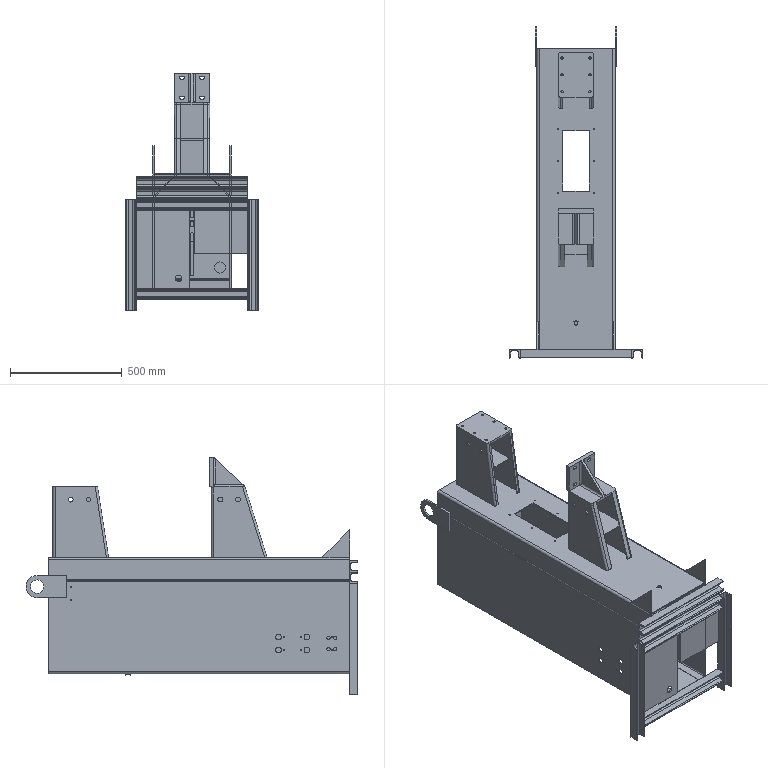Assembly | SolidWorks | mm | 24 component files | 27 solids | 480 faces | box 600 x 1487 x 1065 mm | volume 20129983 mm3 | plane 256 | cylinder 218 | cone 4 | torus 2 | commonest cylinder face diameters 5 x30 10 x27 14 x26 20 x17 7 x14 60 x12 50 x12 10.2 x12
Bill of materials:
001LowerConnectingPlate | 1 | Plain Carbon Steel | Flat rectangular plate, roughly 2:1 aspect ratio, with one large round through-hole and one small round through-hole offset toward one side.
001ReinforcingRib | 2 | Plain Carbon Steel | Thin flat plate with a right-triangle outline (two equal legs at 90 degrees), no visible holes.
001UpperConnectingPlate | 1 | Plain Carbon Steel | Plain flat rectangular plate, roughly 2:1 aspect ratio, with no holes or cutouts.
002FrameBasePanel | 1 | Plain Carbon Steel | Thin flat rectangular plate (portrait proportion) with a single round through-hole near one corner.
002FrameBasePanel2 | 1 | Plain Carbon Steel | Thin flat rectangular plate, slightly wider than tall, with no visible holes or cutouts.
hot-rolled steel channel gb | 6 |  | Straight prismatic channel (C-shaped) profile: a flat web with two flanges whose inner faces taper toward the tips, with filleted inner corners and rounded flange tips.
003FrameFrontWeldingPlate | 1 | Plain Carbon Steel | Bent sheet-metal U-shaped cover/channel: flat top web with two downturned side flanges, a central rectangular cutout, two round holes on either side of it, one small hole near one end, and several tiny point features around the cutout.
004FrameSheet-MetalA | 1 | Plain Carbon Steel | Long bent sheet-metal panel: tall flat web with an inclined top flange and a short bottom return flange, with a small rolled or hooked feature at the bottom bend; a cluster of round holes near one end and two tiny holes near the other end.
005FrameSheet-MetalB | 1 | Plain Carbon Steel | Long bent sheet-metal panel with a tall flat web, an inclined top flange, and a short bottom return flange; one round through-hole and two tiny holes/marks in the web.
006TransformerBasePlate | 1 | Plain Carbon Steel | Sheet-metal bracket plate with chamfered upper corners (pentagon-like outline) and a short bent flange along the bottom edge; four round holes near the corners and two collinear slots along the vertical centerline.
007PartitionPlate | 1 | Plain Carbon Steel | Flat thin plate with chamfered upper corners (pentagon-like outline) and four round through-holes: two near the top and two near the bottom corners.
008FrameTopCoverPlate | 1 | Plain Carbon Steel | Very thin flat rectangular plate (portrait proportion) with slightly rounded corners and two small round holes near the top corners.
009LiftingLug | 2 | Plain Carbon Steel | Flat plate tab of constant thickness. One end is square and the other end is a full semicircle. A single through-hole sits concentric with the rounded end.
010MachineHeadWeldedPart | 1 | Plain Carbon Steel | Formed hollow sheet-metal housing or stand shape. It has a flat top panel with six small holes and side walls that taper and flare outward toward the bottom. Two opposite sides are open below a cross panel, which leaves leg-like wall sections. Each side wall has one larger round hole near the top.
011FrameLowerElectrodeWeldedPart | 1 | Plain Carbon Steel | Bracket with a vertical rectangular mounting flange on top. The flange carries four slotted holes split by a central vertical rib or gusset. The rib slopes down to a tapered, formed channel body with two legs, an internal cross panel, and round holes in the side walls.
hot-rolled equal angle gb | 2 |  | Straight, constant-section angle profile (L-section) with two legs of roughly equal length. It has a root fillet at the inside corner and small rounded tips on the legs. Both ends are cut square.
Mates:
1. distance | 010MachineHeadWeldedPart-1 face at (210, 1367, 320) dir (0, 1, 0) | 011FrameLowerElectrodeWeldedPart-1 face at (210, 657, 320) dir (0, 1, 0)
2. distance | 007PartitionPlate-2 face at (299, 1207, -306) dir (0, 1, 0) | 006TransformerBasePlate-1 face at (-39, 647, -481) dir (0, 1, 0)
3. distance | hot-rolled equal angle gb-1 face at (160, 187, -195) dir (0, -1, 0) | hot-rolled equal angle gb-6 face at (160, 537, -195) dir (0, -1, 0)
4. coincident | 011FrameLowerElectrodeWeldedPart-1 face at (210, 407, 0) dir (0, 0, -1) | 010MachineHeadWeldedPart-1 face at (210, 1117, 0) dir (0, 0, -1)
5. coincident | 011FrameLowerElectrodeWeldedPart-1 face at (50, 667, 320) dir (-1, 0, 0) | 010MachineHeadWeldedPart-1 face at (50, 1367, 0) dir (-1, 0, 0)
6. coincident | 006TransformerBasePlate-1 face at (197.5, 647, -6) dir (0, 0, 1) | 007PartitionPlate-2 face at (62.5, 1202, -6) dir (0, 0, 1)
7. distance | hot-rolled equal angle gb-1 face at (160, 187, -195) dir (0, -1, 0) | 002FrameBaseAssembly-1/002FrameBasePanel-1 face at (-120, 37, -515) dir (0, 1, 0)
8. coincident | hot-rolled equal angle gb-1 face at (-40, 189, -196) dir (-1, 0, 0) | hot-rolled equal angle gb-6 face at (-40, 539, -196) dir (-1, 0, 0)
9. coincident | hot-rolled equal angle gb-1 face at (160, 187, -215) dir (0, 0, -1) | hot-rolled equal angle gb-6 face at (160, 537, -215) dir (0, 0, -1)
10. distance | 006TransformerBasePlate-1 face at (-39, 647, -481) dir (0, 1, 0) | 002FrameBaseAssembly-1/002FrameBasePanel-1 face at (-120, 37, -515) dir (0, 1, 0)
11. coincident | 002FrameBaseAssembly-1/002FrameBasePanel-1 face at (-120, 37, -515) dir (0, 1, 0) | 001LowerConnectingPlate-1 face at (260, 37, -520) dir (0, -1, 0)
12. coincident | 003FrameFrontWeldingPlate-1 face at (-45, 1387, 0) dir (-1, 0, 0) | 001ReinforcingRib-1 face at (-45, 162, 0) dir (-1, 0, 0)
13. coincident | 002FrameBaseAssembly-1/002FrameBasePanel-1 face at (-120, 37, -515) dir (0, 1, 0) | 001ReinforcingRib-1 face at (-45, 37, 0) dir (0, -1, 0)
14. coincident | 003FrameFrontWeldingPlate-1 face at (-45, 1387, 0) dir (0, 0, 1) | 001ReinforcingRib-1 face at (-45, 162, 0) dir (0, 0, -1)
15. distance | 002FrameBaseAssembly-1/hot-rolled steel channel gb-5 face at (420.925, 37, -615) dir (0, 0, -1) | 005FrameSheet-MetalB-1 face at (-105, 1387, -520) dir (0, 0, -1)
16. coincident | 001UpperConnectingPlate-1 face at (260, 1387, -520) dir (0, 0, -1) | 001LowerConnectingPlate-1 face at (0, 162, -520) dir (0, 0, -1)
17. coincident | 004FrameSheet-MetalA-1 face at (0, 1526.253, -4.999) dir (1, 0, 0) | 001LowerConnectingPlate-1 face at (0, 37, -520) dir (-1, 0, 0)
18. coincident | 004FrameSheet-MetalA-1 face at (-40, 1387, -5) dir (1, 0, 0) | hot-rolled equal angle gb-1 face at (-40, 189, -196) dir (-1, 0, 0)
19. distance | 003FrameFrontWeldingPlate-1 face at (-45, 1387, -5) dir (0, 0, -1) | 006TransformerBasePlate-1 face at (197.5, 647, -6) dir (0, 0, 1)
20. distance | hot-rolled equal angle gb-6 edge at (160, 537, -215) dir (-1, 0, 0) | 004FrameSheet-MetalA-1 face at (-45, 1387, -515) dir (0, 0, 1)
21. coincident | 005FrameSheet-MetalB-1 face at (-105, 1387, -520) dir (0, 0, -1) | 001UpperConnectingPlate-1 face at (260, 1387, -520) dir (0, 0, -1)
22. coincident | 005FrameSheet-MetalB-1 face at (305, 1387, -520) dir (0, 1, 0) | 001UpperConnectingPlate-1 face at (0, 1387, -515) dir (0, 1, 0)
23. coincident | 004FrameSheet-MetalA-1 face at (0, 1526.253, -4.999) dir (1, 0, 0) | 001UpperConnectingPlate-1 face at (0, 1247, -515) dir (-1, 0, 0)
24. distance | 008FrameTopCoverPlate-1 face at (299, 1377, -515) dir (0, 1, 0) | 003FrameFrontWeldingPlate-1 face at (305, 1387, -100) dir (0, 1, 0)
25. coincident | 011FrameLowerElectrodeWeldedPart-1 face at (210, 407, 0) dir (0, 0, -1) | 003FrameFrontWeldingPlate-1 face at (-45, 1387, 0) dir (0, 0, 1)
26. width | 010MachineHeadWeldedPart-1 face at (50, 1367, 0) dir (-1, 0, 0) | 010MachineHeadWeldedPart-1 face at (210, 1367, 0) dir (1, 0, 0) | 003FrameFrontWeldingPlate-1 face at (-45, 1387, 0) dir (-1, 0, 0) | 003FrameFrontWeldingPlate-1 face at (305, 1387, 0) dir (1, 0, 0)
27. distance | 011FrameLowerElectrodeWeldedPart-1 face at (210, 657, 320) dir (0, 1, 0) | 002FrameBaseAssembly-1/002FrameBasePanel-1 face at (-120, 37, -515) dir (0, 1, 0)
28. coincident | 003FrameFrontWeldingPlate-1 face at (305, 1387, 0) dir (1, 0, 0) | 001ReinforcingRib-2 face at (305, 162, 0) dir (1, 0, 0)
29. coincident | 002FrameBaseAssembly-1/002FrameBasePanel-1 face at (-120, 37, -515) dir (0, 1, 0) | 001ReinforcingRib-2 face at (297, 37, 0) dir (0, -1, 0)
30. coincident | 003FrameFrontWeldingPlate-1 face at (-45, 1387, 0) dir (0, 0, 1) | 001ReinforcingRib-2 face at (297, 162, 0) dir (0, 0, -1)
31. coincident | 004FrameSheet-MetalA-1 face at (-45, 1387, -5) dir (-1, 0, 0) | 009LiftingLug-1 face at (-45, 1437, -130) dir (1, 0, 0)
32. distance | 009LiftingLug-1 face at (-45, 1437, -80) dir (0, 0, 1) | 003FrameFrontWeldingPlate-1 face at (-45, 1387, 0) dir (0, 0, 1)
33. distance | 009LiftingLug-1 face at (-45, 1307, -80) dir (0, -1, 0) | 003FrameFrontWeldingPlate-1 face at (305, 1387, -100) dir (0, 1, 0)
34. coincident | 005FrameSheet-MetalB-1 face at (305, 1387, -5) dir (1, 0, 0) | 009LiftingLug-2 face at (305, 1437, -130) dir (-1, 0, 0)
35. distance | 009LiftingLug-2 face at (313, 1437, -80) dir (0, 0, 1) | 003FrameFrontWeldingPlate-1 face at (-45, 1387, 0) dir (0, 0, 1)
36. distance | 003FrameFrontWeldingPlate-1 face at (305, 1387, -100) dir (0, 1, 0) | 009LiftingLug-2 face at (313, 1307, -80) dir (0, -1, 0)
37. coincident | 002FrameBaseAssembly-1/002FrameBasePanel-1 face at (-120, 37, -515) dir (0, 1, 0) | 003FrameFrontWeldingPlate-1 face at (305, 37, -100) dir (0, -1, 0)
38. coincident | 005FrameSheet-MetalB-1 face at (305, 1387, -5) dir (1, 0, 0) | 003FrameFrontWeldingPlate-1 face at (305, 1387, 0) dir (1, 0, 0)
39. coincident | 004FrameSheet-MetalA-1 face at (-45, 1387, -5) dir (-1, 0, 0) | 003FrameFrontWeldingPlate-1 face at (-45, 1387, 0) dir (-1, 0, 0)
40. coincident | 004FrameSheet-MetalA-1 face at (365, 37, -520) dir (0, -1, 0) | 005FrameSheet-MetalB-1 face at (305, 37, -520) dir (0, -1, 0)
41. coincident | 002FrameBaseAssembly-1/002FrameBasePanel-1 face at (-120, 37, -515) dir (0, 1, 0) | 004FrameSheet-MetalA-1 face at (365, 37, -520) dir (0, -1, 0)
42. width | 005FrameSheet-MetalB-1 face at (305, 1387, -5) dir (1, 0, 0) | 004FrameSheet-MetalA-1 face at (-45, 1387, -5) dir (-1, 0, 0) | 002FrameBaseAssembly-1/hot-rolled steel channel gb-5 face at (430, 37, -615) dir (1, 0, 0) | 002FrameBaseAssembly-1/hot-rolled steel channel gb-7 face at (-170, 37, -615) dir (-1, 0, 0)
43. distance | 008FrameTopCoverPlate-1 face at (-39, 1372, -5) dir (-1, 0, 0) | 003FrameFrontWeldingPlate-1 face at (-40, 1387, 0) dir (1, 0, 0)
44. coincident | 006TransformerBasePlate-1 face at (299, 647, -107.5) dir (1, 0, 0) | 007PartitionPlate-2 face at (299, 1202, -107.5) dir (1, 0, 0)
45. coincident | 004FrameSheet-MetalA-1 face at (-45, 1387, -520) dir (0, 0, -1) | 005FrameSheet-MetalB-1 face at (-105, 1387, -520) dir (0, 0, -1)
46. coincident | 004FrameSheet-MetalA-1 face at (-45, 1387, -515) dir (0, 0, 1) | 008FrameTopCoverPlate-1 face at (-39, 1372, -515) dir (0, 0, -1)
47. coincident | 003FrameFrontWeldingPlate-1 face at (-45, 1387, 0) dir (0, 0, 1) | assembly plane at (0, 0, 0) dir (0, 0, 1)
48. distance | 005FrameSheet-MetalB-1 face at (-105, 1387, -520) dir (0, 0, -1) | 003FrameFrontWeldingPlate-1 face at (-45, 1387, 0) dir (0, 0, 1)
49. coincident | 002FrameBaseAssembly-1/hot-rolled steel channel gb-5 face at (424.625, 0, -615) dir (0, -1, 0) | assembly plane at (0, 0, 0) dir (0, 1, 0)
50. coincident | 002FrameBaseAssembly-1 plane at (0, 37, -315) dir (1, 0, 0) | assembly plane at (0, 0, 0) dir (1, 0, 0)
51. coincident | 003FrameFrontWeldingPlate-1 plane at (130, 37, -50) dir (1, 0, 0) | 006TransformerBasePlate-1 plane at (130, 642, -481) dir (-1, 0, 0)
52. coincident | hot-rolled steel channel gb-5 face at (300, 0, 380) dir (0, 0, -1) | hot-rolled steel channel gb-6 face at (-159.075, 0, 380) dir (0, 0, 1)
53. coincident | hot-rolled steel channel gb-5 face at (-200, 0, 420.925) dir (-1, 0, 0) | hot-rolled steel channel gb-6 face at (-200, 0, -120) dir (-1, 0, 0)
54. coincident | hot-rolled steel channel gb-6 face at (-200, 0, -120) dir (-1, 0, 0) | hot-rolled steel channel gb-7 face at (-200, 0, -129.075) dir (-1, 0, 0)
55. coincident | hot-rolled steel channel gb-5 face at (300, 0, 380) dir (0, 0, -1) | hot-rolled steel channel gb-8 face at (240.925, 0, 380) dir (0, 0, 1)
56. coincident | hot-rolled steel channel gb-7 face at (300, 0, -120) dir (0, 0, 1) | hot-rolled steel channel gb-9 face at (-209.075, 0, -120) dir (0, 0, -1)
57. coincident | hot-rolled steel channel gb-7 face at (300, 0, -120) dir (0, 0, 1) | hot-rolled steel channel gb-10 face at (-259.075, 0, -120) dir (0, 0, -1)
58. coincident | hot-rolled steel channel gb-9 face at (-250, 0, -120) dir (-1, 0, 0) | hot-rolled steel channel gb-10 face at (-250, 0, -120) dir (1, 0, 0)
59. distance | hot-rolled steel channel gb-9 face at (-200, 0, -120) dir (1, 0, 0) | hot-rolled steel channel gb-8 face at (200, 0, -120) dir (-1, 0, 0)
60. coincident | hot-rolled steel channel gb-6 face at (-150, 0, -120) dir (0, 1, 0) | hot-rolled steel channel gb-7 face at (300, 0, -120) dir (0, 1, 0)
61. coincident | hot-rolled steel channel gb-5 face at (300, 0, 430) dir (0, 1, 0) | hot-rolled steel channel gb-6 face at (-150, 0, -120) dir (0, 1, 0)
62. coincident | hot-rolled steel channel gb-9 face at (-200, 0, -120) dir (0, 1, 0) | hot-rolled steel channel gb-10 face at (-250, 0, -120) dir (0, 1, 0)
63. coincident | hot-rolled steel channel gb-8 face at (250, 0, -120) dir (0, 1, 0) | hot-rolled steel channel gb-9 face at (-200, 0, -120) dir (0, 1, 0)
64. coincident | hot-rolled steel channel gb-6 face at (-150, 0, -120) dir (0, 1, 0) | hot-rolled steel channel gb-10 face at (-250, 0, -120) dir (0, 1, 0)
65. coincident | hot-rolled steel channel gb-6 face at (-159.075, 0, -120) dir (0, 0, -1) | hot-rolled steel channel gb-7 face at (300, 0, -120) dir (0, 0, 1)
66. coincident | 002FrameBasePanel-1 face at (200, 0, -120) dir (0, 1, 0) | hot-rolled steel channel gb-7 face at (300, 0, -120) dir (0, 1, 0)
67. coincident | 002FrameBasePanel-1 face at (-200, -5, -120) dir (0, 0, -1) | hot-rolled steel channel gb-7 face at (300, 0, -120) dir (0, 0, 1)
68. distance | hot-rolled steel channel gb-8 face at (250, 0, -120) dir (1, 0, 0) | hot-rolled steel channel gb-5 face at (300, 0, 420.925) dir (1, 0, 0)
69. coincident | 002FrameBasePanel-1 face at (200, -5, 120) dir (1, 0, 0) | hot-rolled steel channel gb-8 face at (200, 0, -120) dir (-1, 0, 0)
70. coincident | 002FrameBasePanel-1 face at (200, 0, -120) dir (0, 1, 0) | 002FrameBasePanel2-1 face at (45, 0, 140) dir (0, 1, 0)
71. coincident | hot-rolled steel channel gb-5 face at (300, 0, 380) dir (0, 0, -1) | 002FrameBasePanel2-1 face at (-150, -5, 380) dir (0, 0, 1)
72. coincident | hot-rolled steel channel gb-6 face at (-150, 0, -120) dir (1, 0, 0) | 002FrameBasePanel2-1 face at (-150, -5, 380) dir (-1, 0, 0)
73. coincident | 002FrameBasePanel-1 face at (200, 0, -120) dir (0, 1, 0) | 002FrameBaseAssembly plane at (0, 0, 0) dir (0, 1, 0)
74. coincident | 002FrameBasePanel-1 plane at (0, 0, 0) dir (0, 0, 1) | 002FrameBaseAssembly plane at (0, 0, 0) dir (0, 0, 1)
75. coincident | 002FrameBasePanel-1 plane at (0, 0, 0) dir (1, 0, 0) | 002FrameBaseAssembly plane at (0, 0, 0) dir (1, 0, 0)